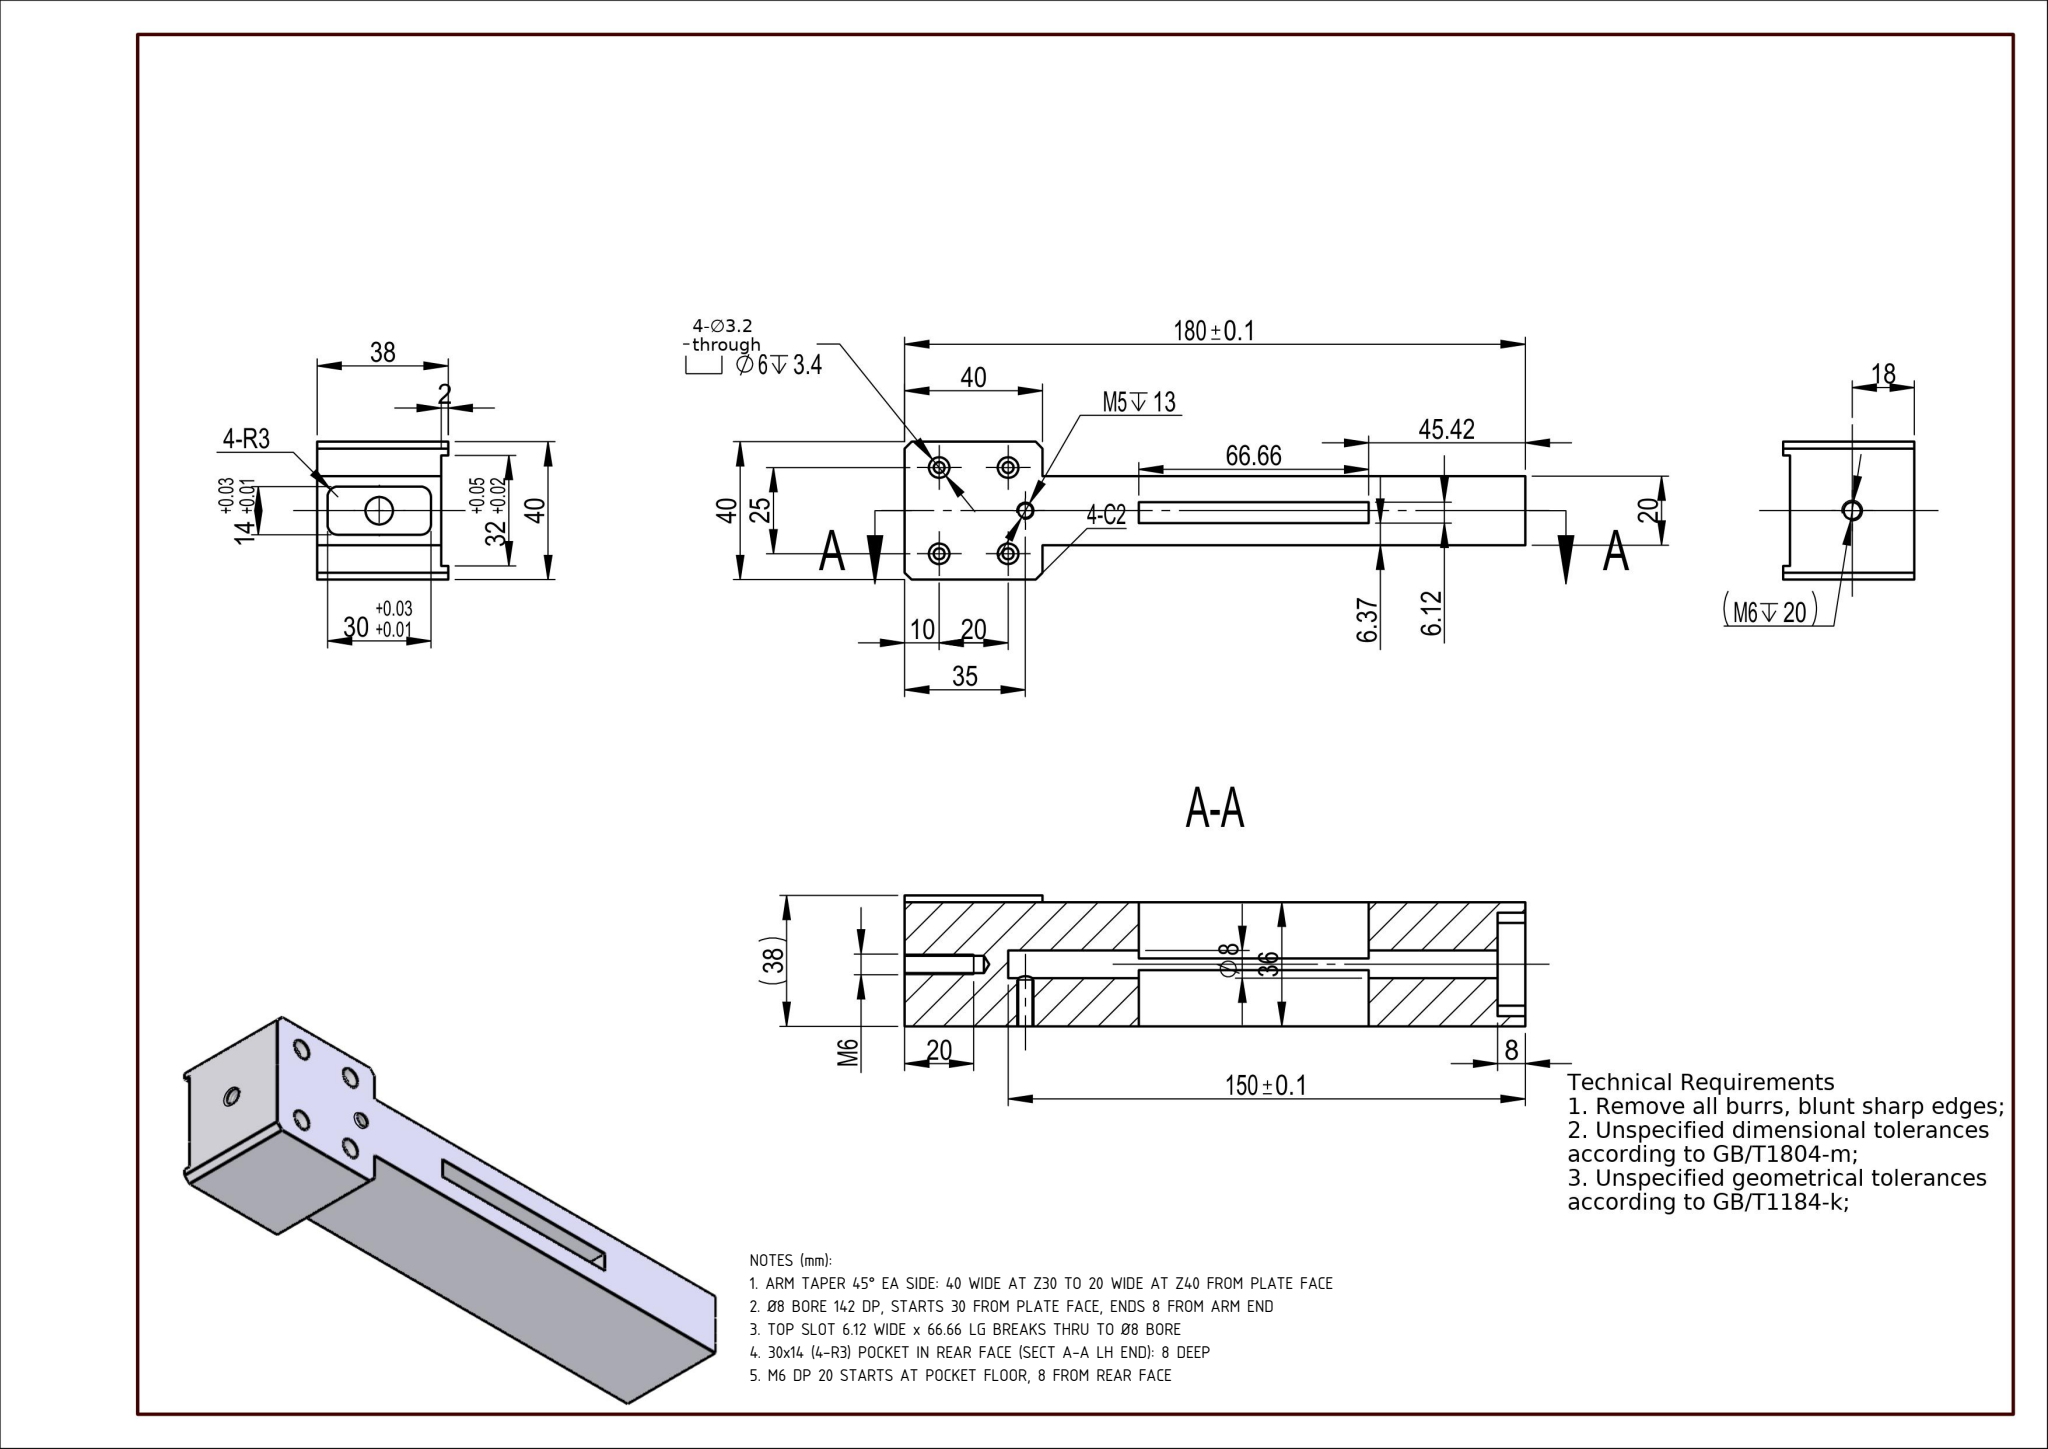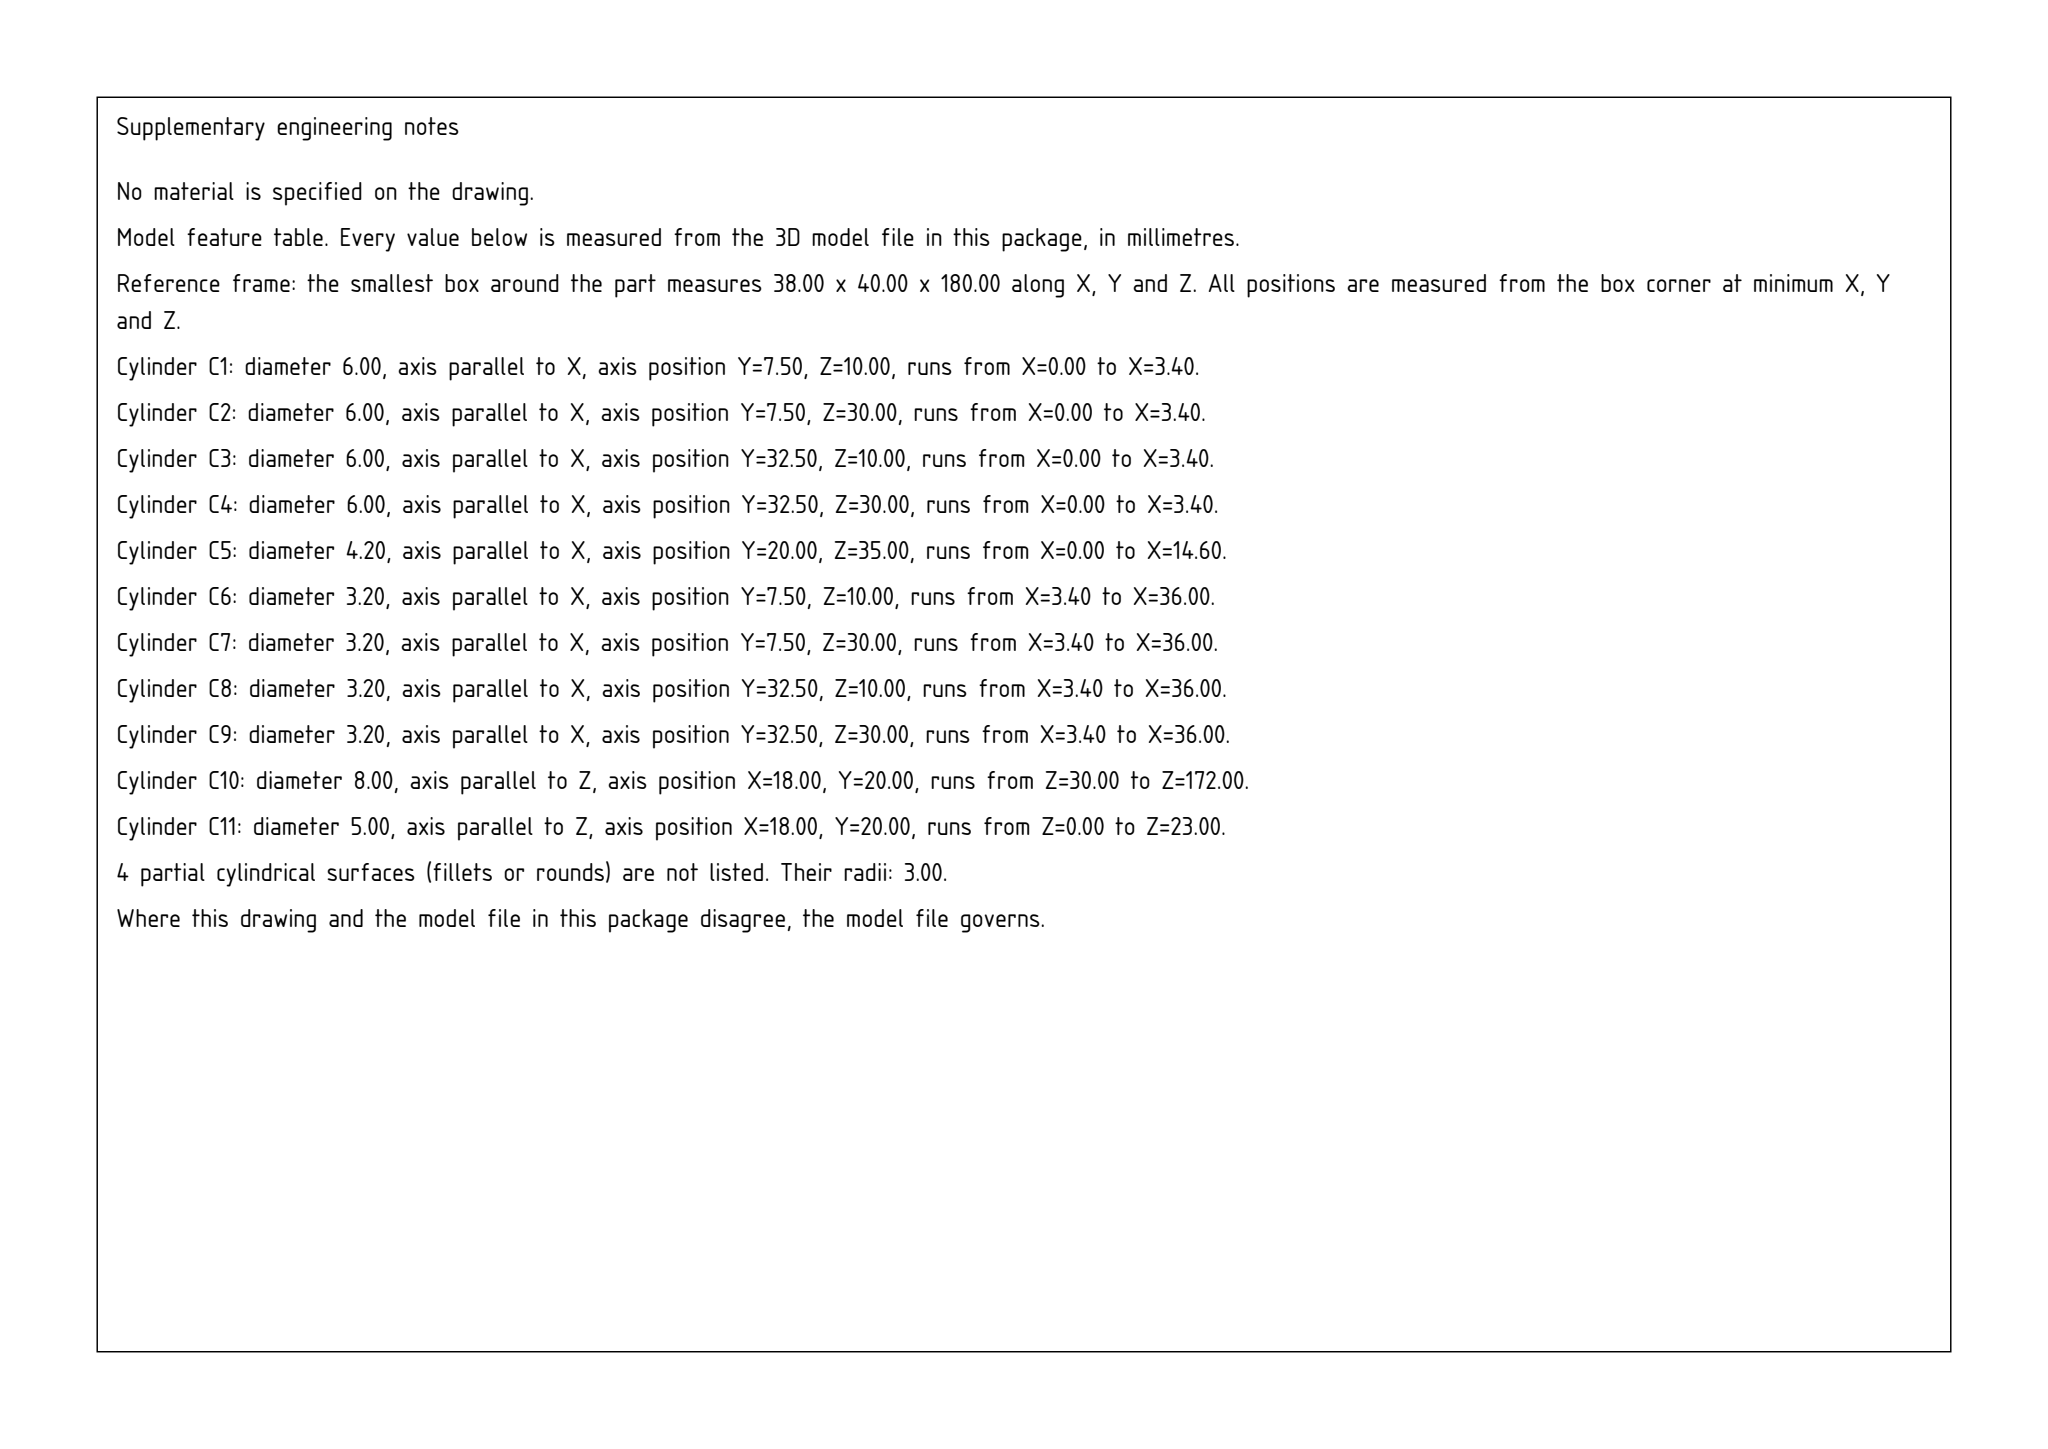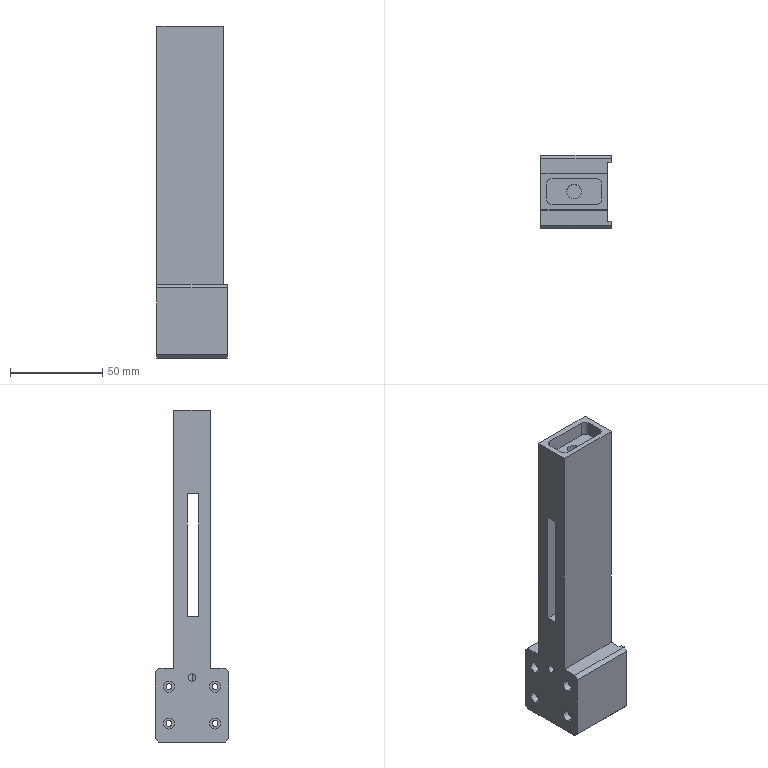Part | SolidWorks | mm | 1 solid | 64 faces | box 38 x 40 x 180 mm | volume 134370 mm3 | plane 36 | cylinder 26 | cone 2 | commonest cylinder face diameters 6 x12 3.2 x8 5 x2 4.2 x2 8 x2
Drawing notes:
ARM TAPER 45° EA SIDE: 40 WIDE AT Z30 TO 20 WIDE AT Z40 FROM PLATE FACE | from the solid: z-plane 30 full width y0-y40; z-plane 40 arm y10-y30 = 20 wide; 10 in z per 10 in y
Ø8 BORE 142 DP, STARTS 30 FROM PLATE FACE, ENDS 8 FROM ARM END | from the solid: cyl Ø8 axis z at x18,y20, L=142, spans z=30 to z=172; z-planes 172 & 180 = 8 to end
TOP SLOT 6.12 WIDE x 66.66 LG BREAKS THRU TO Ø8 BORE | from the solid: y-planes 16.37 & 22.49 = 6.12 wide; z-planes 67.92 & 134.58 = 66.66 lg; same CL as Ø8 bore
30x14 (4-R3) POCKET IN REAR FACE (SECT A-A LH END): 8 DEEP | from the solid: 4x Ø6 z-axis cyls (R3 corners) at x=6/30, y=16/24, length 8 from z=0 face; planes x=3 & x=33 (30 wide), y=13 & y=27 (14 wide)
M6 DP 20 STARTS AT POCKET FLOOR, 8 FROM REAR FACE | from the solid: Ø5 z-axis cyl at (18,20) length 23 starting at pocket floor z=8 (thread 20 deep to z=28, drill point 118°, ref dia 5); Ø8 bore begins z=30
build123d program:
from build123d import *

# Parameters (mm, degrees)
SKETCH1_W                                            = 36
SKETCH1_H                                            = 20
BOSS_EXTRUDE1_DEPTH                                  = 70
SKETCH6_W                                            = 38
SKETCH6_H                                            = 40
BOSS_EXTRUDE2_DEPTH                                  = 40
SKETCH5_W                                            = 30
SKETCH5_H                                            = 14
CUT_EXTRUDE2_DEPTH                                   = 8
SKETCH2_R                                            = 4
CUT_EXTRUDE1_DEPTH                                   = 150
SKETCH7_W                                            = 45
SKETCH7_H                                            = 32
CUT_EXTRUDE3_DEPTH                                   = 2
HOLE_SIZE_ACCORDING_TO_THE_TYPE_OF_HEXAG_D           = 3.2
HOLE_SIZE_ACCORDING_TO_THE_TYPE_OF_HEXAG_CBORE_D     = 6
HOLE_SIZE_ACCORDING_TO_THE_TYPE_OF_HEXAG_CBORE_DEPTH = 3.4
M5_TAPPED_HOLE1_D                                    = 4.2
M5_TAPPED_HOLE1_DEPTH                                = 17.4
M5_TAPPED_HOLE1_TIP                                  = 1.262
FILLET1_R                                            = 3
M6_TAPPED_HOLE1_D                                    = 5
M6_TAPPED_HOLE1_DEPTH                                = 23
M6_TAPPED_HOLE1_TIP                                  = 1.502
CHAMFER1_SIZE                                        = 2
SKETCH13_W                                           = 66.657
SKETCH13_H                                           = 6.124
CUT_EXTRUDE5_DEPTH                                   = 64


with BuildPart() as part:
    # Sketch1 → Boss-Extrude1 (new, symmetric)
    with BuildSketch(Plane.XY):
        Rectangle(SKETCH1_W, SKETCH1_H)
    extrude(amount=BOSS_EXTRUDE1_DEPTH, both=True)

    # Sketch6 → Boss-Extrude2 (add)
    with BuildSketch(Plane(origin=(0, 0, -70), x_dir=(-1, 0, 0), z_dir=(0, 0, -1))):
        with Locations((-1, 0)):
            Rectangle(SKETCH6_W, SKETCH6_H)
    extrude(amount=BOSS_EXTRUDE2_DEPTH)

    # Sketch5 → Cut-Extrude2 (cut)
    with BuildSketch(Plane.XY.offset(70)):
        Rectangle(SKETCH5_W, SKETCH5_H)
    extrude(amount=-CUT_EXTRUDE2_DEPTH, mode=Mode.SUBTRACT)

    # Sketch2 → Cut-Extrude1 (cut)
    with BuildSketch(Plane.XY.offset(70)):
        Circle(SKETCH2_R)
    extrude(amount=-CUT_EXTRUDE1_DEPTH, mode=Mode.SUBTRACT)

    # Sketch7 → Cut-Extrude3 (cut)
    with BuildSketch(Plane(origin=(20, 0, 0), x_dir=(0, 0, -1), z_dir=(1, 0, 0))):
        with Locations((90, 0)):
            Rectangle(SKETCH7_W, SKETCH7_H)
    extrude(amount=-CUT_EXTRUDE3_DEPTH, mode=Mode.SUBTRACT)

    # Hole Size according to the type of hexag (through all)
    with Locations(Plane(origin=(-18, 6.622, 7.557), x_dir=(0, 0, 1), z_dir=(-1, 0, 0))):
        with Locations((-87.557, 5.878), (-87.557, -19.122), (-107.557, -19.122), (-107.557, 5.878)):
            CounterBoreHole(HOLE_SIZE_ACCORDING_TO_THE_TYPE_OF_HEXAG_D / 2, HOLE_SIZE_ACCORDING_TO_THE_TYPE_OF_HEXAG_CBORE_D / 2, HOLE_SIZE_ACCORDING_TO_THE_TYPE_OF_HEXAG_CBORE_DEPTH)

    # M5 Tapped Hole1
    with Locations(Plane.ZY.offset(18)):
        with Locations((-75, 0)):
            Hole(M5_TAPPED_HOLE1_D / 2, depth=M5_TAPPED_HOLE1_DEPTH)
            with Locations((0, 0, -(M5_TAPPED_HOLE1_DEPTH + M5_TAPPED_HOLE1_TIP / 2))):  # 118° drill point
                Cone(0, M5_TAPPED_HOLE1_D / 2, M5_TAPPED_HOLE1_TIP, mode=Mode.SUBTRACT)

    # Fillet1
    fillet1_edges = [part.edges().sort_by_distance(p)[0] for p in [
        (15, 7, 66),
        (15, -7, 66),
        (-15, -7, 66),
        (-15, 7, 66),
    ]]
    fillet(fillet1_edges, radius=FILLET1_R)

    # M6 Tapped Hole1
    with Locations(Plane(origin=(0, 0, -110), x_dir=(-1, 0, 0), z_dir=(0, 0, -1))):
        with Locations((0, 0)):
            Hole(M6_TAPPED_HOLE1_D / 2, depth=M6_TAPPED_HOLE1_DEPTH)
            with Locations((0, 0, -(M6_TAPPED_HOLE1_DEPTH + M6_TAPPED_HOLE1_TIP / 2))):  # 118° drill point
                Cone(0, M6_TAPPED_HOLE1_D / 2, M6_TAPPED_HOLE1_TIP, mode=Mode.SUBTRACT)

    # Chamfer1
    chamfer1_edges = [part.edges().sort_by_distance(p)[0] for p in [
        (1, -20, -70),
        (1, -20, -110),
        (1, 20, -70),
        (1, 20, -110),
    ]]
    chamfer(chamfer1_edges, length=CHAMFER1_SIZE)

    # Sketch13 → Cut-Extrude5 (cut)
    with BuildSketch(Plane(origin=(18, 0, 0), x_dir=(0, 0, -1), z_dir=(1, 0, 0))):
        with Locations((8.748, -0.5697)):
            Rectangle(SKETCH13_W, SKETCH13_H)
    extrude(amount=-CUT_EXTRUDE5_DEPTH, mode=Mode.SUBTRACT)


solid = part.part